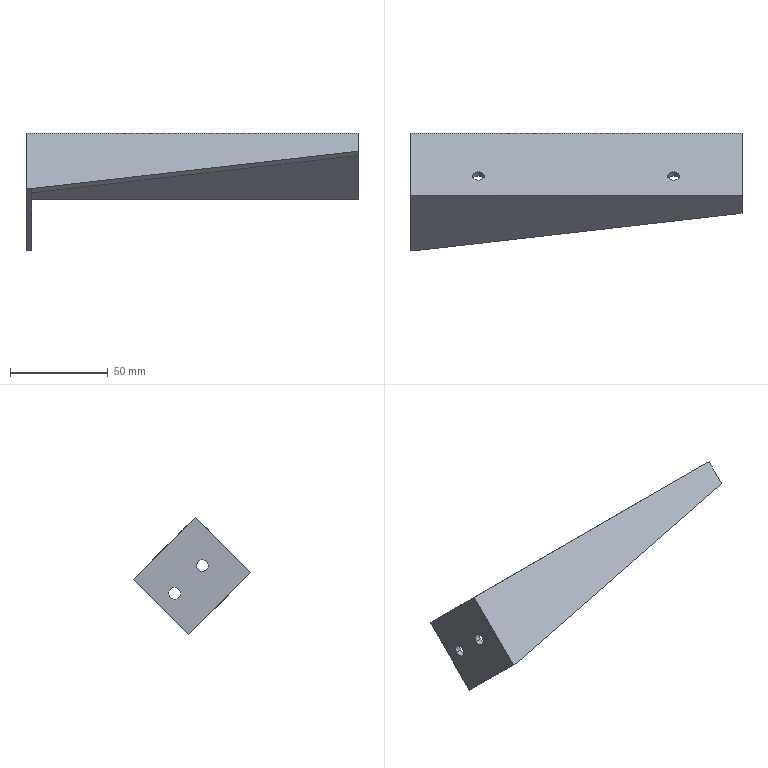Component | SolidWorks | FixedBracket2-1 | 1 solid | 18 faces | box 170 x 60.1 x 60.1 mm | volume 39379 mm3 | plane 10 | cylinder 8 | commonest cylinder face diameters 6 x8
build123d program:
from build123d import *

# Parameters (mm, degrees)
SKETCH1_W           = 45
SKETCH1_H           = 3
EXTRUDE_THIN1_DEPTH = 170
SKETCH2_W           = 45
SKETCH2_H           = 40
BOSS_EXTRUDE1_DEPTH = 3
BOSS_EXTRUDE2_DEPTH = 3
SKETCH4_R           = 3
CUT_EXTRUDE1_DEPTH  = 10
SKETCH5_R           = 3
CUT_EXTRUDE2_DEPTH  = 3


with BuildPart() as part:
    # Sketch1 → Extrude-Thin1 (new body)
    with BuildSketch(Plane.XY):
        with Locations((-41.349, 22.57)):
            Rectangle(SKETCH1_W, SKETCH1_H)
    extrude(amount=EXTRUDE_THIN1_DEPTH)

    # Sketch2 → Boss-Extrude1 (add)
    with BuildSketch(Plane(origin=(0, 0, 0), x_dir=(-1, 0, 0), z_dir=(0, 0, -1))):
        with Locations((41.349, 4.07)):
            Rectangle(SKETCH2_W, SKETCH2_H)
    extrude(amount=-BOSS_EXTRUDE1_DEPTH)

    # Sketch3 → Boss-Extrude2 (add)
    with BuildSketch(Plane.ZY.offset(63.849)):
        Polygon((3, -15.93), (3, 21.07), (170, 21.07), (170, 11.07), align=None)
    extrude(amount=-BOSS_EXTRUDE2_DEPTH)

    # Sketch4 → Cut-Extrude1 (cut)
    with BuildSketch(Plane.XY.offset(3)):
        with Locations((-28.849, 4.07)):
            Circle(SKETCH4_R)
        with Locations((-48.849, 4.07)):
            Circle(SKETCH4_R)
    extrude(amount=-CUT_EXTRUDE1_DEPTH, mode=Mode.SUBTRACT)

    # Sketch5 → Cut-Extrude2 (cut)
    with BuildSketch(Plane(origin=(0, 24.07, 0), x_dir=(1, 0, 0), z_dir=(0, 1, 0))):
        with Locations(Location((-49.849, -35, 0), (0, 0, 270))):
            Circle(SKETCH5_R)
        with Locations(Location((-49.849, -135, 0), (0, 0, 270))):
            Circle(SKETCH5_R)
    extrude(amount=-CUT_EXTRUDE2_DEPTH, mode=Mode.SUBTRACT)


solid = part.part

# Placed as in the assembly
solid = solid.moved(Location((490.45, -365.557, -107.507), (45, 90, 0)))
STEP:
#1=COLOUR_RGB('',0.7922,0.8196,0.9333);
#2=FILL_AREA_STYLE_COLOUR('',#1);
#3=FILL_AREA_STYLE('',(#2));
#4=SURFACE_STYLE_FILL_AREA(#3);
#5=SURFACE_SIDE_STYLE('',(#4));
#6=SURFACE_STYLE_USAGE(.BOTH.,#5);
#7=PRESENTATION_STYLE_ASSIGNMENT((#6));
#8=CARTESIAN_POINT('',(24.506,-15.193,-2.258));
#9=VERTEX_POINT('',#8);
#10=CARTESIAN_POINT('',(24.742,-15.193,-2.258));
#11=VERTEX_POINT('',#10);
#12=CARTESIAN_POINT('',(24.624,-15.193,-2.258));
#13=DIRECTION('',(0.,0.7071,0.7071));
#14=DIRECTION('',(1.,0.,0.));
#15=AXIS2_PLACEMENT_3D('',#12,#13,#14);
#16=CIRCLE('',#15,0.1181);
#17=EDGE_CURVE('',#9,#11,#16,.T.);
#18=ORIENTED_EDGE('',*,*,#17,.F.);
#19=CARTESIAN_POINT('',(24.506,-15.11,-2.175));
#20=VERTEX_POINT('',#19);
#21=CARTESIAN_POINT('',(24.506,-15.193,-2.258));
#22=DIRECTION('',(0.,0.7071,0.7071));
#23=VECTOR('',#22,39.37);
#24=LINE('',#21,#23);
#25=EDGE_CURVE('',#9,#20,#24,.T.);
#26=ORIENTED_EDGE('',*,*,#25,.T.);
#27=CARTESIAN_POINT('',(24.742,-15.11,-2.175));
#28=VERTEX_POINT('',#27);
#29=CARTESIAN_POINT('',(24.624,-15.11,-2.175));
#30=DIRECTION('',(0.,0.7071,0.7071));
#31=DIRECTION('',(1.,0.,0.));
#32=AXIS2_PLACEMENT_3D('',#29,#30,#31);
#33=CIRCLE('',#32,0.1181);
#34=EDGE_CURVE('',#20,#28,#33,.T.);
#35=ORIENTED_EDGE('',*,*,#34,.T.);
#36=CARTESIAN_POINT('',(24.742,-15.193,-2.258));
#37=DIRECTION('',(0.,0.7071,0.7071));
#38=VECTOR('',#37,39.37);
#39=LINE('',#36,#38);
#40=EDGE_CURVE('',#11,#28,#39,.T.);
#41=ORIENTED_EDGE('',*,*,#40,.F.);
#42=EDGE_LOOP('',(#18,#26,#35,#41));
#43=FACE_OUTER_BOUND('',#42,.T.);
#44=CARTESIAN_POINT('',(24.624,-15.193,-2.258));
#45=DIRECTION('',(0.,0.7071,0.7071));
#46=DIRECTION('',(1.,0.,0.));
#47=AXIS2_PLACEMENT_3D('',#44,#45,#46);
#48=CYLINDRICAL_SURFACE('',#47,0.1181);
#49=ADVANCED_FACE('',(#43),#48,.F.);
#50=CARTESIAN_POINT('',(20.569,-15.193,-2.258));
#51=VERTEX_POINT('',#50);
#52=CARTESIAN_POINT('',(20.805,-15.193,-2.258));
#53=VERTEX_POINT('',#52);
#54=CARTESIAN_POINT('',(20.687,-15.193,-2.258));
#55=DIRECTION('',(0.,0.7071,0.7071));
#56=DIRECTION('',(1.,0.,0.));
#57=AXIS2_PLACEMENT_3D('',#54,#55,#56);
#58=CIRCLE('',#57,0.1181);
#59=EDGE_CURVE('',#51,#53,#58,.T.);
#60=ORIENTED_EDGE('',*,*,#59,.F.);
#61=CARTESIAN_POINT('',(20.569,-15.11,-2.175));
#62=VERTEX_POINT('',#61);
#63=CARTESIAN_POINT('',(20.569,-15.193,-2.258));
#64=DIRECTION('',(0.,0.7071,0.7071));
#65=VECTOR('',#64,39.37);
#66=LINE('',#63,#65);
#67=EDGE_CURVE('',#51,#62,#66,.T.);
#68=ORIENTED_EDGE('',*,*,#67,.T.);
#69=CARTESIAN_POINT('',(20.805,-15.11,-2.175));
#70=VERTEX_POINT('',#69);
#71=CARTESIAN_POINT('',(20.687,-15.11,-2.175));
#72=DIRECTION('',(0.,0.7071,0.7071));
#73=DIRECTION('',(1.,0.,0.));
#74=AXIS2_PLACEMENT_3D('',#71,#72,#73);
#75=CIRCLE('',#74,0.1181);
#76=EDGE_CURVE('',#62,#70,#75,.T.);
#77=ORIENTED_EDGE('',*,*,#76,.T.);
#78=CARTESIAN_POINT('',(20.805,-15.193,-2.258));
#79=DIRECTION('',(0.,0.7071,0.7071));
#80=VECTOR('',#79,39.37);
#81=LINE('',#78,#80);
#82=EDGE_CURVE('',#53,#70,#81,.T.);
#83=ORIENTED_EDGE('',*,*,#82,.F.);
#84=EDGE_LOOP('',(#60,#68,#77,#83));
#85=FACE_OUTER_BOUND('',#84,.T.);
#86=CARTESIAN_POINT('',(20.687,-15.193,-2.258));
#87=DIRECTION('',(0.,0.7071,0.7071));
#88=DIRECTION('',(1.,0.,0.));
#89=AXIS2_PLACEMENT_3D('',#86,#87,#88);
#90=CYLINDRICAL_SURFACE('',#89,0.1181);
#91=ADVANCED_FACE('',(#85),#90,.F.);
#92=CARTESIAN_POINT('',(19.309,-15.555,-2.843));
#93=VERTEX_POINT('',#92);
#94=CARTESIAN_POINT('',(19.309,-15.722,-2.676));
#95=VERTEX_POINT('',#94);
#96=CARTESIAN_POINT('',(19.309,-15.639,-2.759));
#97=DIRECTION('',(-1.,-0.,0.));
#98=DIRECTION('',(0.,-0.7071,0.7071));
#99=AXIS2_PLACEMENT_3D('',#96,#97,#98);
#100=CIRCLE('',#99,0.1181);
#101=EDGE_CURVE('',#93,#95,#100,.T.);
#102=ORIENTED_EDGE('',*,*,#101,.T.);
#103=CARTESIAN_POINT('',(19.427,-15.722,-2.676));
#104=VERTEX_POINT('',#103);
#105=CARTESIAN_POINT('',(19.033,-15.722,-2.676));
#106=DIRECTION('',(1.,0.,-0.));
#107=VECTOR('',#106,39.37);
#108=LINE('',#105,#107);
#109=EDGE_CURVE('',#95,#104,#108,.T.);
#110=ORIENTED_EDGE('',*,*,#109,.T.);
#111=CARTESIAN_POINT('',(19.427,-15.555,-2.843));
#112=VERTEX_POINT('',#111);
#113=CARTESIAN_POINT('',(19.427,-15.639,-2.759));
#114=DIRECTION('',(1.,0.,-0.));
#115=DIRECTION('',(0.,0.7071,-0.7071));
#116=AXIS2_PLACEMENT_3D('',#113,#114,#115);
#117=CIRCLE('',#116,0.1181);
#118=EDGE_CURVE('',#104,#112,#117,.T.);
#119=ORIENTED_EDGE('',*,*,#118,.T.);
#120=CARTESIAN_POINT('',(19.033,-15.555,-2.843));
#121=DIRECTION('',(1.,0.,-0.));
#122=VECTOR('',#121,39.37);
#123=LINE('',#120,#122);
#124=EDGE_CURVE('',#93,#112,#123,.T.);
#125=ORIENTED_EDGE('',*,*,#124,.F.);
#126=EDGE_LOOP('',(#102,#110,#119,#125));
#127=FACE_OUTER_BOUND('',#126,.T.);
#128=CARTESIAN_POINT('',(19.033,-15.639,-2.759));
#129=DIRECTION('',(1.,0.,-0.));
#130=DIRECTION('',(0.,0.7071,-0.7071));
#131=AXIS2_PLACEMENT_3D('',#128,#129,#130);
#132=CYLINDRICAL_SURFACE('',#131,0.1181);
#133=ADVANCED_FACE('',(#127),#132,.F.);
#134=CARTESIAN_POINT('',(19.309,-14.998,-3.4));
#135=VERTEX_POINT('',#134);
#136=CARTESIAN_POINT('',(19.309,-15.165,-3.233));
#137=VERTEX_POINT('',#136);
#138=CARTESIAN_POINT('',(19.309,-15.082,-3.316));
#139=DIRECTION('',(-1.,-0.,0.));
#140=DIRECTION('',(0.,-0.7071,0.7071));
#141=AXIS2_PLACEMENT_3D('',#138,#139,#140);
#142=CIRCLE('',#141,0.1181);
#143=EDGE_CURVE('',#135,#137,#142,.T.);
#144=ORIENTED_EDGE('',*,*,#143,.T.);
#145=CARTESIAN_POINT('',(19.427,-15.165,-3.233));
#146=VERTEX_POINT('',#145);
#147=CARTESIAN_POINT('',(19.033,-15.165,-3.233));
#148=DIRECTION('',(1.,0.,-0.));
#149=VECTOR('',#148,39.37);
#150=LINE('',#147,#149);
#151=EDGE_CURVE('',#137,#146,#150,.T.);
#152=ORIENTED_EDGE('',*,*,#151,.T.);
#153=CARTESIAN_POINT('',(19.427,-14.998,-3.4));
#154=VERTEX_POINT('',#153);
#155=CARTESIAN_POINT('',(19.427,-15.082,-3.316));
#156=DIRECTION('',(1.,0.,-0.));
#157=DIRECTION('',(0.,0.7071,-0.7071));
#158=AXIS2_PLACEMENT_3D('',#155,#156,#157);
#159=CIRCLE('',#158,0.1181);
#160=EDGE_CURVE('',#146,#154,#159,.T.);
#161=ORIENTED_EDGE('',*,*,#160,.T.);
#162=CARTESIAN_POINT('',(19.033,-14.998,-3.4));
#163=DIRECTION('',(1.,0.,-0.));
#164=VECTOR('',#163,39.37);
#165=LINE('',#162,#164);
#166=EDGE_CURVE('',#135,#154,#165,.T.);
#167=ORIENTED_EDGE('',*,*,#166,.F.);
#168=EDGE_LOOP('',(#144,#152,#161,#167));
#169=FACE_OUTER_BOUND('',#168,.T.);
#170=CARTESIAN_POINT('',(19.033,-15.082,-3.316));
#171=DIRECTION('',(1.,0.,-0.));
#172=DIRECTION('',(0.,0.7071,-0.7071));
#173=AXIS2_PLACEMENT_3D('',#170,#171,#172);
#174=CYLINDRICAL_SURFACE('',#173,0.1181);
#175=ADVANCED_FACE('',(#169),#174,.F.);
#176=CARTESIAN_POINT('',(24.624,-15.193,-2.258));
#177=DIRECTION('',(0.,0.7071,0.7071));
#178=DIRECTION('',(1.,0.,0.));
#179=AXIS2_PLACEMENT_3D('',#176,#177,#178);
#180=CIRCLE('',#179,0.1181);
#181=EDGE_CURVE('',#11,#9,#180,.T.);
#182=ORIENTED_EDGE('',*,*,#181,.T.);
#183=ORIENTED_EDGE('',*,*,#17,.T.);
#184=EDGE_LOOP('',(#182,#183));
#185=FACE_BOUND('',#184,.T.);
#186=CARTESIAN_POINT('',(20.687,-15.193,-2.258));
#187=DIRECTION('',(0.,0.7071,0.7071));
#188=DIRECTION('',(1.,0.,0.));
#189=AXIS2_PLACEMENT_3D('',#186,#187,#188);
#190=CIRCLE('',#189,0.1181);
#191=EDGE_CURVE('',#53,#51,#190,.T.);
#192=ORIENTED_EDGE('',*,*,#191,.T.);
#193=ORIENTED_EDGE('',*,*,#59,.T.);
#194=EDGE_LOOP('',(#192,#193));
#195=FACE_BOUND('',#194,.T.);
#196=CARTESIAN_POINT('',(26.002,-15.499,-1.952));
#197=VERTEX_POINT('',#196);
#198=CARTESIAN_POINT('',(26.002,-14.33,-3.121));
#199=VERTEX_POINT('',#198);
#200=CARTESIAN_POINT('',(26.002,-15.583,-1.869));
#201=DIRECTION('',(0.,0.7071,-0.7071));
#202=VECTOR('',#201,39.37);
#203=LINE('',#200,#202);
#204=EDGE_CURVE('',#197,#199,#203,.T.);
#205=ORIENTED_EDGE('',*,*,#204,.F.);
#206=CARTESIAN_POINT('',(19.427,-15.499,-1.952));
#207=VERTEX_POINT('',#206);
#208=CARTESIAN_POINT('',(19.427,-15.499,-1.952));
#209=DIRECTION('',(-1.,-0.,0.));
#210=VECTOR('',#209,39.37);
#211=LINE('',#208,#210);
#212=EDGE_CURVE('',#197,#207,#211,.T.);
#213=ORIENTED_EDGE('',*,*,#212,.T.);
#214=CARTESIAN_POINT('',(19.427,-14.33,-3.121));
#215=VERTEX_POINT('',#214);
#216=CARTESIAN_POINT('',(19.427,-15.583,-1.869));
#217=DIRECTION('',(-0.,-0.7071,0.7071));
#218=VECTOR('',#217,39.37);
#219=LINE('',#216,#218);
#220=EDGE_CURVE('',#215,#207,#219,.T.);
#221=ORIENTED_EDGE('',*,*,#220,.F.);
#222=CARTESIAN_POINT('',(26.002,-14.33,-3.121));
#223=DIRECTION('',(-1.,-0.,0.));
#224=VECTOR('',#223,39.37);
#225=LINE('',#222,#224);
#226=EDGE_CURVE('',#199,#215,#225,.T.);
#227=ORIENTED_EDGE('',*,*,#226,.F.);
#228=EDGE_LOOP('',(#205,#213,#221,#227));
#229=FACE_OUTER_BOUND('',#228,.T.);
#230=CARTESIAN_POINT('',(26.002,-15.583,-1.869));
#231=DIRECTION('',(-0.,0.7071,0.7071));
#232=DIRECTION('',(1.,0.,-0.));
#233=AXIS2_PLACEMENT_3D('',#230,#231,#232);
#234=PLANE('',#233);
#235=ADVANCED_FACE('',(#185,#195,#229),#234,.F.);
#236=CARTESIAN_POINT('',(19.309,-14.247,-3.038));
#237=VERTEX_POINT('',#236);
#238=CARTESIAN_POINT('',(19.309,-15.36,-4.151));
#239=VERTEX_POINT('',#238);
#240=CARTESIAN_POINT('',(19.309,-14.247,-3.038));
#241=DIRECTION('',(-0.,-0.7071,-0.7071));
#242=VECTOR('',#241,39.37);
#243=LINE('',#240,#242);
#244=EDGE_CURVE('',#237,#239,#243,.T.);
#245=ORIENTED_EDGE('',*,*,#244,.F.);
#246=CARTESIAN_POINT('',(26.002,-14.247,-3.038));
#247=VERTEX_POINT('',#246);
#248=CARTESIAN_POINT('',(26.002,-14.247,-3.038));
#249=DIRECTION('',(-1.,-0.,0.));
#250=VECTOR('',#249,39.37);
#251=LINE('',#248,#250);
#252=EDGE_CURVE('',#247,#237,#251,.T.);
#253=ORIENTED_EDGE('',*,*,#252,.F.);
#254=CARTESIAN_POINT('',(26.002,-14.247,-3.038));
#255=DIRECTION('',(-0.,-0.7071,-0.7071));
#256=VECTOR('',#255,39.37);
#257=LINE('',#254,#256);
#258=EDGE_CURVE('',#247,#199,#257,.T.);
#259=ORIENTED_EDGE('',*,*,#258,.T.);
#260=ORIENTED_EDGE('',*,*,#226,.T.);
#261=CARTESIAN_POINT('',(19.427,-15.36,-4.151));
#262=VERTEX_POINT('',#261);
#263=CARTESIAN_POINT('',(19.427,-14.247,-3.038));
#264=DIRECTION('',(-0.,-0.7071,-0.7071));
#265=VECTOR('',#264,39.37);
#266=LINE('',#263,#265);
#267=EDGE_CURVE('',#215,#262,#266,.T.);
#268=ORIENTED_EDGE('',*,*,#267,.T.);
#269=CARTESIAN_POINT('',(19.427,-15.36,-4.151));
#270=DIRECTION('',(-1.,-0.,0.));
#271=VECTOR('',#270,39.37);
#272=LINE('',#269,#271);
#273=EDGE_CURVE('',#262,#239,#272,.T.);
#274=ORIENTED_EDGE('',*,*,#273,.T.);
#275=EDGE_LOOP('',(#245,#253,#259,#260,#268,#274));
#276=FACE_OUTER_BOUND('',#275,.T.);
#277=CARTESIAN_POINT('',(26.002,-14.247,-3.038));
#278=DIRECTION('',(-0.,0.7071,-0.7071));
#279=DIRECTION('',(-1.,-0.,0.));
#280=AXIS2_PLACEMENT_3D('',#277,#278,#279);
#281=PLANE('',#280);
#282=ADVANCED_FACE('',(#276),#281,.T.);
#283=CARTESIAN_POINT('',(24.624,-15.11,-2.175));
#284=DIRECTION('',(0.,0.7071,0.7071));
#285=DIRECTION('',(1.,0.,0.));
#286=AXIS2_PLACEMENT_3D('',#283,#284,#285);
#287=CIRCLE('',#286,0.1181);
#288=EDGE_CURVE('',#28,#20,#287,.T.);
#289=ORIENTED_EDGE('',*,*,#288,.F.);
#290=ORIENTED_EDGE('',*,*,#34,.F.);
#291=EDGE_LOOP('',(#289,#290));
#292=FACE_BOUND('',#291,.T.);
#293=CARTESIAN_POINT('',(20.687,-15.11,-2.175));
#294=DIRECTION('',(0.,0.7071,0.7071));
#295=DIRECTION('',(1.,0.,0.));
#296=AXIS2_PLACEMENT_3D('',#293,#294,#295);
#297=CIRCLE('',#296,0.1181);
#298=EDGE_CURVE('',#70,#62,#297,.T.);
#299=ORIENTED_EDGE('',*,*,#298,.F.);
#300=ORIENTED_EDGE('',*,*,#76,.F.);
#301=EDGE_LOOP('',(#299,#300));
#302=FACE_BOUND('',#301,.T.);
#303=CARTESIAN_POINT('',(19.309,-15.499,-1.785));
#304=VERTEX_POINT('',#303);
#305=CARTESIAN_POINT('',(19.309,-15.499,-1.785));
#306=DIRECTION('',(0.,0.7071,-0.7071));
#307=VECTOR('',#306,39.37);
#308=LINE('',#305,#307);
#309=EDGE_CURVE('',#304,#237,#308,.T.);
#310=ORIENTED_EDGE('',*,*,#309,.F.);
#311=CARTESIAN_POINT('',(26.002,-15.499,-1.785));
#312=VERTEX_POINT('',#311);
#313=CARTESIAN_POINT('',(26.002,-15.499,-1.785));
#314=DIRECTION('',(-1.,-0.,0.));
#315=VECTOR('',#314,39.37);
#316=LINE('',#313,#315);
#317=EDGE_CURVE('',#312,#304,#316,.T.);
#318=ORIENTED_EDGE('',*,*,#317,.F.);
#319=CARTESIAN_POINT('',(26.002,-15.499,-1.785));
#320=DIRECTION('',(0.,0.7071,-0.7071));
#321=VECTOR('',#320,39.37);
#322=LINE('',#319,#321);
#323=EDGE_CURVE('',#312,#247,#322,.T.);
#324=ORIENTED_EDGE('',*,*,#323,.T.);
#325=ORIENTED_EDGE('',*,*,#252,.T.);
#326=EDGE_LOOP('',(#310,#318,#324,#325));
#327=FACE_OUTER_BOUND('',#326,.T.);
#328=CARTESIAN_POINT('',(26.002,-15.499,-1.785));
#329=DIRECTION('',(-0.,0.7071,0.7071));
#330=DIRECTION('',(1.,0.,-0.));
#331=AXIS2_PLACEMENT_3D('',#328,#329,#330);
#332=PLANE('',#331);
#333=ADVANCED_FACE('',(#292,#302,#327),#332,.T.);
#334=CARTESIAN_POINT('',(19.309,-16.613,-2.899));
#335=VERTEX_POINT('',#334);
#336=CARTESIAN_POINT('',(19.309,-15.583,-1.869));
#337=DIRECTION('',(0.,0.7071,0.7071));
#338=VECTOR('',#337,39.37);
#339=LINE('',#336,#338);
#340=EDGE_CURVE('',#335,#304,#339,.T.);
#341=ORIENTED_EDGE('',*,*,#340,.F.);
#342=CARTESIAN_POINT('',(19.427,-16.613,-2.899));
#343=VERTEX_POINT('',#342);
#344=CARTESIAN_POINT('',(19.427,-16.613,-2.899));
#345=DIRECTION('',(-1.,-0.,0.));
#346=VECTOR('',#345,39.37);
#347=LINE('',#344,#346);
#348=EDGE_CURVE('',#343,#335,#347,.T.);
#349=ORIENTED_EDGE('',*,*,#348,.F.);
#350=CARTESIAN_POINT('',(26.002,-15.861,-2.147));
#351=VERTEX_POINT('',#350);
#352=CARTESIAN_POINT('',(26.002,-15.861,-2.147));
#353=DIRECTION('',(0.9872,0.1129,0.1129));
#354=VECTOR('',#353,39.37);
#355=LINE('',#352,#354);
#356=EDGE_CURVE('',#343,#351,#355,.T.);
#357=ORIENTED_EDGE('',*,*,#356,.T.);
#358=CARTESIAN_POINT('',(26.002,-15.583,-1.869));
#359=DIRECTION('',(0.,0.7071,0.7071));
#360=VECTOR('',#359,39.37);
#361=LINE('',#358,#360);
#362=EDGE_CURVE('',#351,#312,#361,.T.);
#363=ORIENTED_EDGE('',*,*,#362,.T.);
#364=ORIENTED_EDGE('',*,*,#317,.T.);
#365=EDGE_LOOP('',(#341,#349,#357,#363,#364));
#366=FACE_OUTER_BOUND('',#365,.T.);
#367=CARTESIAN_POINT('',(26.002,-15.583,-1.869));
#368=DIRECTION('',(0.,-0.7071,0.7071));
#369=DIRECTION('',(1.,0.,-0.));
#370=AXIS2_PLACEMENT_3D('',#367,#368,#369);
#371=PLANE('',#370);
#372=ADVANCED_FACE('',(#366),#371,.T.);
#373=ORIENTED_EDGE('',*,*,#362,.F.);
#374=CARTESIAN_POINT('',(26.002,-15.778,-2.23));
#375=VERTEX_POINT('',#374);
#376=CARTESIAN_POINT('',(26.002,-15.778,-2.23));
#377=DIRECTION('',(-0.,-0.7071,0.7071));
#378=VECTOR('',#377,39.37);
#379=LINE('',#376,#378);
#380=EDGE_CURVE('',#375,#351,#379,.T.);
#381=ORIENTED_EDGE('',*,*,#380,.F.);
#382=CARTESIAN_POINT('',(26.002,-15.499,-1.952));
#383=DIRECTION('',(0.,0.7071,0.7071));
#384=VECTOR('',#383,39.37);
#385=LINE('',#382,#384);
#386=EDGE_CURVE('',#375,#197,#385,.T.);
#387=ORIENTED_EDGE('',*,*,#386,.T.);
#388=ORIENTED_EDGE('',*,*,#204,.T.);
#389=ORIENTED_EDGE('',*,*,#258,.F.);
#390=ORIENTED_EDGE('',*,*,#323,.F.);
#391=EDGE_LOOP('',(#373,#381,#387,#388,#389,#390));
#392=FACE_OUTER_BOUND('',#391,.T.);
#393=CARTESIAN_POINT('',(26.002,-14.392,-4.233));
#394=DIRECTION('',(-1.,-0.,-0.));
#395=DIRECTION('',(-0.,-0.7071,0.7071));
#396=AXIS2_PLACEMENT_3D('',#393,#394,#395);
#397=PLANE('',#396);
#398=ADVANCED_FACE('',(#392),#397,.F.);
#399=ORIENTED_EDGE('',*,*,#101,.F.);
#400=CARTESIAN_POINT('',(19.309,-15.639,-2.759));
#401=DIRECTION('',(-1.,-0.,0.));
#402=DIRECTION('',(0.,-0.7071,0.7071));
#403=AXIS2_PLACEMENT_3D('',#400,#401,#402);
#404=CIRCLE('',#403,0.1181);
#405=EDGE_CURVE('',#95,#93,#404,.T.);
#406=ORIENTED_EDGE('',*,*,#405,.F.);
#407=EDGE_LOOP('',(#399,#406));
#408=FACE_BOUND('',#407,.T.);
#409=ORIENTED_EDGE('',*,*,#143,.F.);
#410=CARTESIAN_POINT('',(19.309,-15.082,-3.316));
#411=DIRECTION('',(-1.,-0.,0.));
#412=DIRECTION('',(0.,-0.7071,0.7071));
#413=AXIS2_PLACEMENT_3D('',#410,#411,#412);
#414=CIRCLE('',#413,0.1181);
#415=EDGE_CURVE('',#137,#135,#414,.T.);
#416=ORIENTED_EDGE('',*,*,#415,.F.);
#417=EDGE_LOOP('',(#409,#416));
#418=FACE_BOUND('',#417,.T.);
#419=ORIENTED_EDGE('',*,*,#244,.T.);
#420=CARTESIAN_POINT('',(19.309,-15.36,-4.151));
#421=DIRECTION('',(-0.,-0.7071,0.7071));
#422=VECTOR('',#421,39.37);
#423=LINE('',#420,#422);
#424=EDGE_CURVE('',#239,#335,#423,.T.);
#425=ORIENTED_EDGE('',*,*,#424,.T.);
#426=ORIENTED_EDGE('',*,*,#340,.T.);
#427=ORIENTED_EDGE('',*,*,#309,.T.);
#428=EDGE_LOOP('',(#419,#425,#426,#427));
#429=FACE_OUTER_BOUND('',#428,.T.);
#430=CARTESIAN_POINT('',(19.309,-14.392,-4.233));
#431=DIRECTION('',(-1.,-0.,-0.));
#432=DIRECTION('',(-0.,-0.7071,0.7071));
#433=AXIS2_PLACEMENT_3D('',#430,#431,#432);
#434=PLANE('',#433);
#435=ADVANCED_FACE('',(#408,#418,#429),#434,.T.);
#436=CARTESIAN_POINT('',(19.427,-15.639,-2.759));
#437=DIRECTION('',(1.,0.,-0.));
#438=DIRECTION('',(0.,0.7071,-0.7071));
#439=AXIS2_PLACEMENT_3D('',#436,#437,#438);
#440=CIRCLE('',#439,0.1181);
#441=EDGE_CURVE('',#112,#104,#440,.T.);
#442=ORIENTED_EDGE('',*,*,#441,.F.);
#443=ORIENTED_EDGE('',*,*,#118,.F.);
#444=EDGE_LOOP('',(#442,#443));
#445=FACE_BOUND('',#444,.T.);
#446=CARTESIAN_POINT('',(19.427,-15.082,-3.316));
#447=DIRECTION('',(1.,0.,-0.));
#448=DIRECTION('',(0.,0.7071,-0.7071));
#449=AXIS2_PLACEMENT_3D('',#446,#447,#448);
#450=CIRCLE('',#449,0.1181);
#451=EDGE_CURVE('',#154,#146,#450,.T.);
#452=ORIENTED_EDGE('',*,*,#451,.F.);
#453=ORIENTED_EDGE('',*,*,#160,.F.);
#454=EDGE_LOOP('',(#452,#453));
#455=FACE_BOUND('',#454,.T.);
#456=ORIENTED_EDGE('',*,*,#220,.T.);
#457=CARTESIAN_POINT('',(19.427,-16.529,-2.982));
#458=VERTEX_POINT('',#457);
#459=CARTESIAN_POINT('',(19.427,-16.529,-2.982));
#460=DIRECTION('',(-0.,-0.7071,-0.7071));
#461=VECTOR('',#460,39.37);
#462=LINE('',#459,#461);
#463=EDGE_CURVE('',#207,#458,#462,.T.);
#464=ORIENTED_EDGE('',*,*,#463,.T.);
#465=CARTESIAN_POINT('',(19.427,-15.36,-4.151));
#466=DIRECTION('',(-0.,-0.7071,0.7071));
#467=VECTOR('',#466,39.37);
#468=LINE('',#465,#467);
#469=EDGE_CURVE('',#262,#458,#468,.T.);
#470=ORIENTED_EDGE('',*,*,#469,.F.);
#471=ORIENTED_EDGE('',*,*,#267,.F.);
#472=EDGE_LOOP('',(#456,#464,#470,#471));
#473=FACE_OUTER_BOUND('',#472,.T.);
#474=CARTESIAN_POINT('',(19.427,-14.392,-4.233));
#475=DIRECTION('',(-1.,-0.,-0.));
#476=DIRECTION('',(-0.,-0.7071,0.7071));
#477=AXIS2_PLACEMENT_3D('',#474,#475,#476);
#478=PLANE('',#477);
#479=ADVANCED_FACE('',(#445,#455,#473),#478,.F.);
#480=ORIENTED_EDGE('',*,*,#424,.F.);
#481=ORIENTED_EDGE('',*,*,#273,.F.);
#482=ORIENTED_EDGE('',*,*,#469,.T.);
#483=CARTESIAN_POINT('',(19.427,-16.529,-2.982));
#484=DIRECTION('',(-0.,-0.7071,0.7071));
#485=VECTOR('',#484,39.37);
#486=LINE('',#483,#485);
#487=EDGE_CURVE('',#458,#343,#486,.T.);
#488=ORIENTED_EDGE('',*,*,#487,.T.);
#489=ORIENTED_EDGE('',*,*,#348,.T.);
#490=EDGE_LOOP('',(#480,#481,#482,#488,#489));
#491=FACE_OUTER_BOUND('',#490,.T.);
#492=CARTESIAN_POINT('',(19.427,-15.36,-4.151));
#493=DIRECTION('',(0.,-0.7071,-0.7071));
#494=DIRECTION('',(-1.,-0.,0.));
#495=AXIS2_PLACEMENT_3D('',#492,#493,#494);
#496=PLANE('',#495);
#497=ADVANCED_FACE('',(#491),#496,.T.);
#498=ORIENTED_EDGE('',*,*,#356,.F.);
#499=ORIENTED_EDGE('',*,*,#487,.F.);
#500=CARTESIAN_POINT('',(26.002,-15.778,-2.23));
#501=DIRECTION('',(0.9872,0.1129,0.1129));
#502=VECTOR('',#501,39.37);
#503=LINE('',#500,#502);
#504=EDGE_CURVE('',#458,#375,#503,.T.);
#505=ORIENTED_EDGE('',*,*,#504,.T.);
#506=ORIENTED_EDGE('',*,*,#380,.T.);
#507=EDGE_LOOP('',(#498,#499,#505,#506));
#508=FACE_OUTER_BOUND('',#507,.T.);
#509=CARTESIAN_POINT('',(26.002,-15.778,-2.23));
#510=DIRECTION('',(0.1596,-0.698,-0.698));
#511=DIRECTION('',(-0.9872,-0.1129,-0.1129));
#512=AXIS2_PLACEMENT_3D('',#509,#510,#511);
#513=PLANE('',#512);
#514=ADVANCED_FACE('',(#508),#513,.T.);
#515=ORIENTED_EDGE('',*,*,#504,.F.);
#516=ORIENTED_EDGE('',*,*,#463,.F.);
#517=ORIENTED_EDGE('',*,*,#212,.F.);
#518=ORIENTED_EDGE('',*,*,#386,.F.);
#519=EDGE_LOOP('',(#515,#516,#517,#518));
#520=FACE_OUTER_BOUND('',#519,.T.);
#521=CARTESIAN_POINT('',(19.309,-16.086,-2.539));
#522=DIRECTION('',(-0.,0.7071,-0.7071));
#523=DIRECTION('',(-1.,-0.,0.));
#524=AXIS2_PLACEMENT_3D('',#521,#522,#523);
#525=PLANE('',#524);
#526=ADVANCED_FACE('',(#520),#525,.T.);
#527=ORIENTED_EDGE('',*,*,#151,.F.);
#528=ORIENTED_EDGE('',*,*,#415,.T.);
#529=ORIENTED_EDGE('',*,*,#166,.T.);
#530=ORIENTED_EDGE('',*,*,#451,.T.);
#531=EDGE_LOOP('',(#527,#528,#529,#530));
#532=FACE_OUTER_BOUND('',#531,.T.);
#533=CARTESIAN_POINT('',(19.033,-15.082,-3.316));
#534=DIRECTION('',(1.,0.,-0.));
#535=DIRECTION('',(0.,0.7071,-0.7071));
#536=AXIS2_PLACEMENT_3D('',#533,#534,#535);
#537=CYLINDRICAL_SURFACE('',#536,0.1181);
#538=ADVANCED_FACE('',(#532),#537,.F.);
#539=ORIENTED_EDGE('',*,*,#109,.F.);
#540=ORIENTED_EDGE('',*,*,#405,.T.);
#541=ORIENTED_EDGE('',*,*,#124,.T.);
#542=ORIENTED_EDGE('',*,*,#441,.T.);
#543=EDGE_LOOP('',(#539,#540,#541,#542));
#544=FACE_OUTER_BOUND('',#543,.T.);
#545=CARTESIAN_POINT('',(19.033,-15.639,-2.759));
#546=DIRECTION('',(1.,0.,-0.));
#547=DIRECTION('',(0.,0.7071,-0.7071));
#548=AXIS2_PLACEMENT_3D('',#545,#546,#547);
#549=CYLINDRICAL_SURFACE('',#548,0.1181);
#550=ADVANCED_FACE('',(#544),#549,.F.);
#551=ORIENTED_EDGE('',*,*,#67,.F.);
#552=ORIENTED_EDGE('',*,*,#191,.F.);
#553=ORIENTED_EDGE('',*,*,#82,.T.);
#554=ORIENTED_EDGE('',*,*,#298,.T.);
#555=EDGE_LOOP('',(#551,#552,#553,#554));
#556=FACE_OUTER_BOUND('',#555,.T.);
#557=CARTESIAN_POINT('',(20.687,-15.193,-2.258));
#558=DIRECTION('',(0.,0.7071,0.7071));
#559=DIRECTION('',(1.,0.,0.));
#560=AXIS2_PLACEMENT_3D('',#557,#558,#559);
#561=CYLINDRICAL_SURFACE('',#560,0.1181);
#562=ADVANCED_FACE('',(#556),#561,.F.);
#563=ORIENTED_EDGE('',*,*,#25,.F.);
#564=ORIENTED_EDGE('',*,*,#181,.F.);
#565=ORIENTED_EDGE('',*,*,#40,.T.);
#566=ORIENTED_EDGE('',*,*,#288,.T.);
#567=EDGE_LOOP('',(#563,#564,#565,#566));
#568=FACE_OUTER_BOUND('',#567,.T.);
#569=CARTESIAN_POINT('',(24.624,-15.193,-2.258));
#570=DIRECTION('',(0.,0.7071,0.7071));
#571=DIRECTION('',(1.,0.,0.));
#572=AXIS2_PLACEMENT_3D('',#569,#570,#571);
#573=CYLINDRICAL_SURFACE('',#572,0.1181);
#574=ADVANCED_FACE('',(#568),#573,.F.);
#575=CLOSED_SHELL('',(#49,#91,#133,#175,#235,#282,#333,#372,#398,#435,#479,#497,#514,#526,#538,#550,#562,#574));
#576=MANIFOLD_SOLID_BREP('',#575);
#577=STYLED_ITEM('',(#7),#576);
#578=PRESENTATION_LAYER_ASSIGNMENT('','',(#577));
#579=(LENGTH_UNIT()NAMED_UNIT(*)SI_UNIT($,.METRE.));
#580=LENGTH_MEASURE_WITH_UNIT(LENGTH_MEASURE(0.0254),#579);
#581=DIMENSIONAL_EXPONENTS(1.,0.,0.,0.,0.,0.,0.);
#582=(CONVERSION_BASED_UNIT('',#580)LENGTH_UNIT()NAMED_UNIT(#581));
#583=UNCERTAINTY_MEASURE_WITH_UNIT(LENGTH_MEASURE(0.00001),#582,'','');
#584=(NAMED_UNIT(*)PLANE_ANGLE_UNIT()SI_UNIT($,.RADIAN.));
#585=(NAMED_UNIT(*)SI_UNIT($,.STERADIAN.)SOLID_ANGLE_UNIT());
#586=(GEOMETRIC_REPRESENTATION_CONTEXT(3)GLOBAL_UNCERTAINTY_ASSIGNED_CONTEXT((#583))GLOBAL_UNIT_ASSIGNED_CONTEXT((#582,#584,#585))REPRESENTATION_CONTEXT('',''));
#587=MECHANICAL_DESIGN_GEOMETRIC_PRESENTATION_REPRESENTATION('',(#577),#586);
#588=CARTESIAN_POINT('',(0.,0.,0.));
#589=DIRECTION('',(0.,0.,1.));
#590=DIRECTION('',(1.,0.,0.));
#591=AXIS2_PLACEMENT_3D('',#588,#589,#590);
#592=(LENGTH_UNIT()NAMED_UNIT(*)SI_UNIT($,.METRE.));
#593=LENGTH_MEASURE_WITH_UNIT(LENGTH_MEASURE(0.0254),#592);
#594=DIMENSIONAL_EXPONENTS(1.,0.,0.,0.,0.,0.,0.);
#595=(CONVERSION_BASED_UNIT('',#593)LENGTH_UNIT()NAMED_UNIT(#594));
#596=UNCERTAINTY_MEASURE_WITH_UNIT(LENGTH_MEASURE(0.00001),#595,'','');
#597=(NAMED_UNIT(*)PLANE_ANGLE_UNIT()SI_UNIT($,.RADIAN.));
#598=(NAMED_UNIT(*)SI_UNIT($,.STERADIAN.)SOLID_ANGLE_UNIT());
#599=(GEOMETRIC_REPRESENTATION_CONTEXT(3)GLOBAL_UNCERTAINTY_ASSIGNED_CONTEXT((#596))GLOBAL_UNIT_ASSIGNED_CONTEXT((#595,#597,#598))REPRESENTATION_CONTEXT('',''));
#600=ADVANCED_BREP_SHAPE_REPRESENTATION('',(#576,#591),#599);